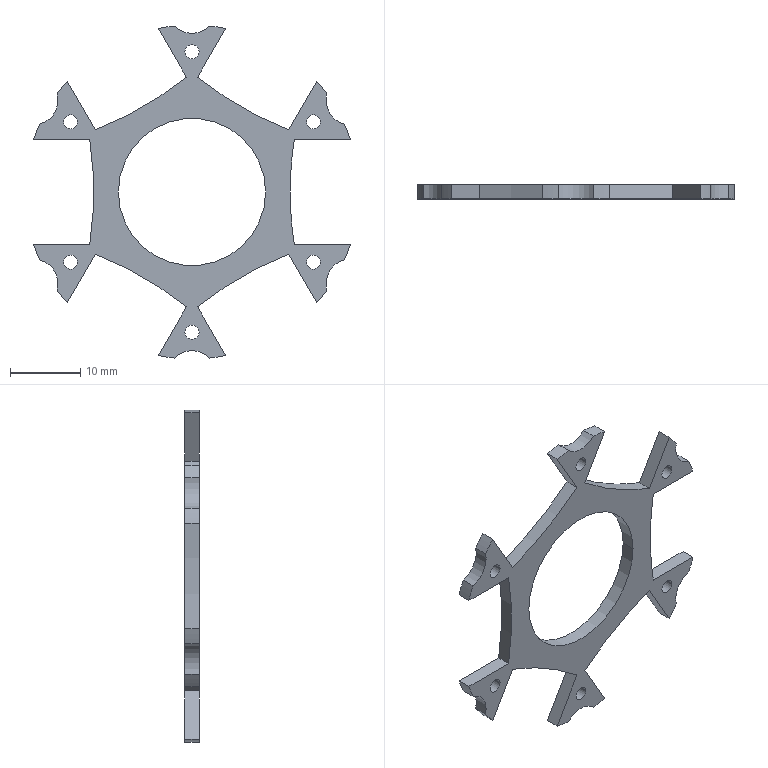Component | SolidWorks | Half-1_SidePlate-1 | 1 solid | 55 faces | box 45.17 x 2 x 47.34 mm | volume 1123 mm3 | cylinder 41 | plane 14 | commonest cylinder face diameters 2 x12 47.6 x12 7 x8 96.351 x7 21 x2 | material 1060 Alloy
build123d program:
from build123d import *

# Parameters (mm, degrees)
SKETCH1_R           = 1
SKETCH1_R_2         = 10.5
BOSS_EXTRUDE1_DEPTH = 2


with BuildPart() as part:
    # Sketch1 → Boss-Extrude1 (new body)
    with BuildSketch(Plane.XY):
        with BuildLine():
            ThreePointArc((13.789, 8.883), (7, 12.124), (0.7985, 16.383))
            Line((0.7985, 16.383), (4.799, 23.311))
            ThreePointArc((4.799, 23.311), (3.654, 23.518), (2.5, 23.668))
            ThreePointArc((2.5, 23.668), (0, 22.618), (-2.5, 23.668))
            ThreePointArc((-2.5, 23.668), (-3.654, 23.518), (-4.799, 23.311))
            Line((-4.799, 23.311), (-0.7985, 16.383))
            ThreePointArc((-0.7985, 16.383), (-7, 12.124), (-13.789, 8.883))
            Line((-13.789, 8.883), (-17.789, 15.811))
            ThreePointArc((-17.789, 15.811), (-18.54, 14.923), (-19.247, 13.999))
            ThreePointArc((-19.247, 13.999), (-19.588, 11.309), (-21.747, 9.669))
            ThreePointArc((-21.747, 9.669), (-22.194, 8.595), (-22.587, 7.5))
            Line((-22.587, 7.5), (-14.587, 7.5))
            ThreePointArc((-14.587, 7.5), (-14, 0), (-14.587, -7.5))
            Line((-14.587, -7.5), (-22.587, -7.5))
            ThreePointArc((-22.587, -7.5), (-22.194, -8.595), (-21.747, -9.669))
            ThreePointArc((-21.747, -9.669), (-19.588, -11.309), (-19.247, -13.999))
            ThreePointArc((-19.247, -13.999), (-18.54, -14.923), (-17.789, -15.811))
            Line((-17.789, -15.811), (-13.789, -8.883))
            ThreePointArc((-13.789, -8.883), (-7, -12.124), (-0.7985, -16.383))
            Line((-0.7985, -16.383), (-4.799, -23.311))
            ThreePointArc((-4.799, -23.311), (-3.654, -23.518), (-2.5, -23.668))
            ThreePointArc((-2.5, -23.668), (0, -22.618), (2.5, -23.668))
            ThreePointArc((2.5, -23.668), (3.654, -23.518), (4.799, -23.311))
            Line((4.799, -23.311), (0.7985, -16.383))
            ThreePointArc((0.7985, -16.383), (7, -12.124), (13.789, -8.883))
            Line((13.789, -8.883), (17.789, -15.811))
            ThreePointArc((17.789, -15.811), (18.54, -14.923), (19.247, -13.999))
            ThreePointArc((19.247, -13.999), (19.588, -11.309), (21.747, -9.669))
            ThreePointArc((21.747, -9.669), (22.194, -8.595), (22.587, -7.5))
            Line((22.587, -7.5), (14.587, -7.5))
            ThreePointArc((14.587, -7.5), (14, 0), (14.587, 7.5))
            Line((14.587, 7.5), (22.587, 7.5))
            ThreePointArc((22.587, 7.5), (22.194, 8.595), (21.747, 9.669))
            ThreePointArc((21.747, 9.669), (19.588, 11.309), (19.247, 13.999))
            ThreePointArc((19.247, 13.999), (18.54, 14.923), (17.789, 15.811))
            Line((17.789, 15.811), (13.789, 8.883))
        make_face()
        with Locations((-17.321, -10)):
            Circle(SKETCH1_R, mode=Mode.SUBTRACT)
        with Locations((0, -20)):
            Circle(SKETCH1_R, mode=Mode.SUBTRACT)
        with Locations((17.321, -10)):
            Circle(SKETCH1_R, mode=Mode.SUBTRACT)
        with Locations((-17.321, 10)):
            Circle(SKETCH1_R, mode=Mode.SUBTRACT)
        Circle(SKETCH1_R_2, mode=Mode.SUBTRACT)
        with Locations((17.321, 10)):
            Circle(SKETCH1_R, mode=Mode.SUBTRACT)
        with Locations((0, 20)):
            Circle(SKETCH1_R, mode=Mode.SUBTRACT)
    extrude(amount=BOSS_EXTRUDE1_DEPTH)


solid = part.part

# Placed as in the assembly
solid = solid.moved(Location((0.3183, 1.4, 37), (90, 0, 0)))